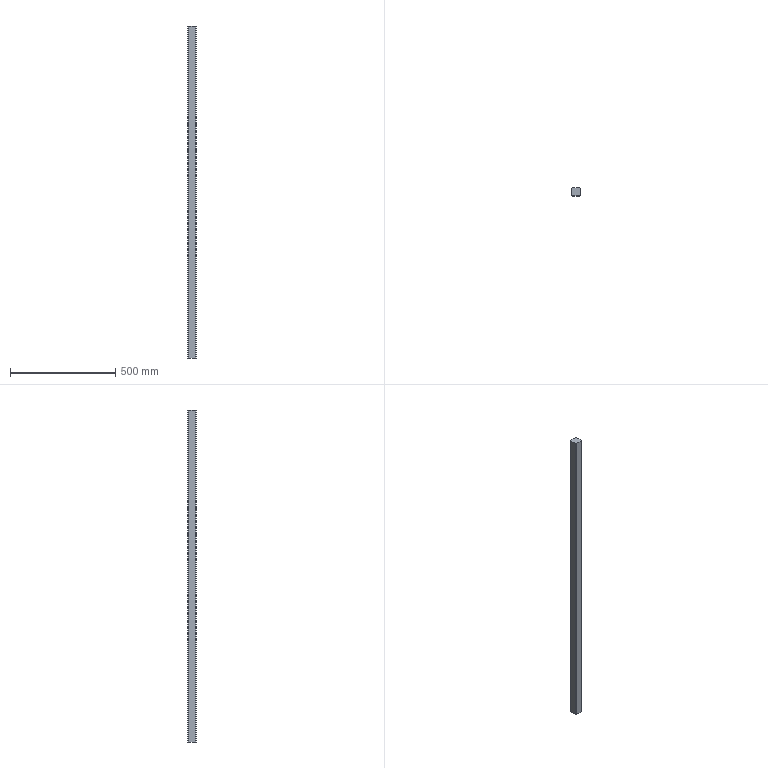Component | SolidWorks | Jig4040-1580-2 | 1 solid | 10 faces | box 40 x 40 x 1580 mm | volume 2494093 mm3 | plane 6 | cylinder 4 | commonest cylinder face diameters 10 x4 | material Copper
build123d program:
from build123d import *

# Parameters (mm, degrees)
SKETCH1_W           = 40
SKETCH1_H           = 40
BOSS_EXTRUDE1_DEPTH = 1580
FILLET1_R           = 5


with BuildPart() as part:
    # Sketch1 → Boss-Extrude1 (new body)
    with BuildSketch(Plane.XY):
        with Locations((20, 20)):
            Rectangle(SKETCH1_W, SKETCH1_H)
    extrude(amount=BOSS_EXTRUDE1_DEPTH)

    # Fillet1
    fillet1_edges = [part.edges().sort_by_distance(p)[0] for p in [
        (0, 40, 790),
        (40, 40, 790),
        (40, 0, 790),
        (0, 0, 790),
    ]]
    fillet(fillet1_edges, radius=FILLET1_R)


solid = part.part

# Placed as in the assembly
solid = solid.moved(Location((711.992, -17.909, 790), (0, 0, 0)))
STEP:
#1=CARTESIAN_POINT('',(28.031,0.6729,31.102));
#2=VERTEX_POINT('',#1);
#3=CARTESIAN_POINT('',(28.031,-0.5082,31.102));
#4=VERTEX_POINT('',#3);
#5=CARTESIAN_POINT('',(28.031,-0.7051,31.102));
#6=DIRECTION('',(0.,-1.,0.));
#7=VECTOR('',#6,39.37);
#8=LINE('',#5,#7);
#9=EDGE_CURVE('',#2,#4,#8,.T.);
#10=ORIENTED_EDGE('',*,*,#9,.T.);
#11=CARTESIAN_POINT('',(28.031,-0.5082,93.307));
#12=VERTEX_POINT('',#11);
#13=CARTESIAN_POINT('',(28.031,-0.5082,93.307));
#14=DIRECTION('',(0.,0.,1.));
#15=VECTOR('',#14,39.37);
#16=LINE('',#13,#15);
#17=EDGE_CURVE('',#4,#12,#16,.T.);
#18=ORIENTED_EDGE('',*,*,#17,.T.);
#19=CARTESIAN_POINT('',(28.031,0.6729,93.307));
#20=VERTEX_POINT('',#19);
#21=CARTESIAN_POINT('',(28.031,-0.7051,93.307));
#22=DIRECTION('',(0.,-1.,0.));
#23=VECTOR('',#22,39.37);
#24=LINE('',#21,#23);
#25=EDGE_CURVE('',#20,#12,#24,.T.);
#26=ORIENTED_EDGE('',*,*,#25,.F.);
#27=CARTESIAN_POINT('',(28.031,0.6729,93.307));
#28=DIRECTION('',(0.,0.,-1.));
#29=VECTOR('',#28,39.37);
#30=LINE('',#27,#29);
#31=EDGE_CURVE('',#20,#2,#30,.T.);
#32=ORIENTED_EDGE('',*,*,#31,.T.);
#33=EDGE_LOOP('',(#10,#18,#26,#32));
#34=FACE_OUTER_BOUND('',#33,.T.);
#35=CARTESIAN_POINT('',(28.031,-0.7051,93.307));
#36=DIRECTION('',(1.,0.,0.));
#37=DIRECTION('',(0.,0.,-1.));
#38=AXIS2_PLACEMENT_3D('',#35,#36,#37);
#39=PLANE('',#38);
#40=ADVANCED_FACE('',(#34),#39,.F.);
#41=CARTESIAN_POINT('',(28.228,-0.7051,93.307));
#42=VERTEX_POINT('',#41);
#43=CARTESIAN_POINT('',(29.409,-0.7051,93.307));
#44=VERTEX_POINT('',#43);
#45=CARTESIAN_POINT('',(28.031,-0.7051,93.307));
#46=DIRECTION('',(1.,0.,0.));
#47=VECTOR('',#46,39.37);
#48=LINE('',#45,#47);
#49=EDGE_CURVE('',#42,#44,#48,.T.);
#50=ORIENTED_EDGE('',*,*,#49,.F.);
#51=CARTESIAN_POINT('',(28.228,-0.7051,31.102));
#52=VERTEX_POINT('',#51);
#53=CARTESIAN_POINT('',(28.228,-0.7051,93.307));
#54=DIRECTION('',(0.,0.,-1.));
#55=VECTOR('',#54,39.37);
#56=LINE('',#53,#55);
#57=EDGE_CURVE('',#42,#52,#56,.T.);
#58=ORIENTED_EDGE('',*,*,#57,.T.);
#59=CARTESIAN_POINT('',(29.409,-0.7051,31.102));
#60=VERTEX_POINT('',#59);
#61=CARTESIAN_POINT('',(28.031,-0.7051,31.102));
#62=DIRECTION('',(1.,0.,0.));
#63=VECTOR('',#62,39.37);
#64=LINE('',#61,#63);
#65=EDGE_CURVE('',#52,#60,#64,.T.);
#66=ORIENTED_EDGE('',*,*,#65,.T.);
#67=CARTESIAN_POINT('',(29.409,-0.7051,93.307));
#68=DIRECTION('',(0.,0.,1.));
#69=VECTOR('',#68,39.37);
#70=LINE('',#67,#69);
#71=EDGE_CURVE('',#60,#44,#70,.T.);
#72=ORIENTED_EDGE('',*,*,#71,.T.);
#73=EDGE_LOOP('',(#50,#58,#66,#72));
#74=FACE_OUTER_BOUND('',#73,.T.);
#75=CARTESIAN_POINT('',(28.031,-0.7051,93.307));
#76=DIRECTION('',(0.,1.,0.));
#77=DIRECTION('',(0.,0.,1.));
#78=AXIS2_PLACEMENT_3D('',#75,#76,#77);
#79=PLANE('',#78);
#80=ADVANCED_FACE('',(#74),#79,.F.);
#81=CARTESIAN_POINT('',(29.606,-0.5082,93.307));
#82=VERTEX_POINT('',#81);
#83=CARTESIAN_POINT('',(29.606,0.6729,93.307));
#84=VERTEX_POINT('',#83);
#85=CARTESIAN_POINT('',(29.606,-0.7051,93.307));
#86=DIRECTION('',(0.,1.,0.));
#87=VECTOR('',#86,39.37);
#88=LINE('',#85,#87);
#89=EDGE_CURVE('',#82,#84,#88,.T.);
#90=ORIENTED_EDGE('',*,*,#89,.F.);
#91=CARTESIAN_POINT('',(29.606,-0.5082,31.102));
#92=VERTEX_POINT('',#91);
#93=CARTESIAN_POINT('',(29.606,-0.5082,93.307));
#94=DIRECTION('',(0.,0.,-1.));
#95=VECTOR('',#94,39.37);
#96=LINE('',#93,#95);
#97=EDGE_CURVE('',#82,#92,#96,.T.);
#98=ORIENTED_EDGE('',*,*,#97,.T.);
#99=CARTESIAN_POINT('',(29.606,0.6729,31.102));
#100=VERTEX_POINT('',#99);
#101=CARTESIAN_POINT('',(29.606,-0.7051,31.102));
#102=DIRECTION('',(0.,1.,0.));
#103=VECTOR('',#102,39.37);
#104=LINE('',#101,#103);
#105=EDGE_CURVE('',#92,#100,#104,.T.);
#106=ORIENTED_EDGE('',*,*,#105,.T.);
#107=CARTESIAN_POINT('',(29.606,0.6729,93.307));
#108=DIRECTION('',(0.,0.,1.));
#109=VECTOR('',#108,39.37);
#110=LINE('',#107,#109);
#111=EDGE_CURVE('',#100,#84,#110,.T.);
#112=ORIENTED_EDGE('',*,*,#111,.T.);
#113=EDGE_LOOP('',(#90,#98,#106,#112));
#114=FACE_OUTER_BOUND('',#113,.T.);
#115=CARTESIAN_POINT('',(29.606,-0.7051,93.307));
#116=DIRECTION('',(-1.,0.,0.));
#117=DIRECTION('',(0.,0.,1.));
#118=AXIS2_PLACEMENT_3D('',#115,#116,#117);
#119=PLANE('',#118);
#120=ADVANCED_FACE('',(#114),#119,.F.);
#121=CARTESIAN_POINT('',(29.409,0.8697,31.102));
#122=VERTEX_POINT('',#121);
#123=CARTESIAN_POINT('',(28.228,0.8697,31.102));
#124=VERTEX_POINT('',#123);
#125=CARTESIAN_POINT('',(28.031,0.8697,31.102));
#126=DIRECTION('',(-1.,0.,0.));
#127=VECTOR('',#126,39.37);
#128=LINE('',#125,#127);
#129=EDGE_CURVE('',#122,#124,#128,.T.);
#130=ORIENTED_EDGE('',*,*,#129,.T.);
#131=CARTESIAN_POINT('',(28.228,0.8697,93.307));
#132=VERTEX_POINT('',#131);
#133=CARTESIAN_POINT('',(28.228,0.8697,93.307));
#134=DIRECTION('',(0.,0.,1.));
#135=VECTOR('',#134,39.37);
#136=LINE('',#133,#135);
#137=EDGE_CURVE('',#124,#132,#136,.T.);
#138=ORIENTED_EDGE('',*,*,#137,.T.);
#139=CARTESIAN_POINT('',(29.409,0.8697,93.307));
#140=VERTEX_POINT('',#139);
#141=CARTESIAN_POINT('',(28.031,0.8697,93.307));
#142=DIRECTION('',(-1.,0.,0.));
#143=VECTOR('',#142,39.37);
#144=LINE('',#141,#143);
#145=EDGE_CURVE('',#140,#132,#144,.T.);
#146=ORIENTED_EDGE('',*,*,#145,.F.);
#147=CARTESIAN_POINT('',(29.409,0.8697,93.307));
#148=DIRECTION('',(0.,0.,-1.));
#149=VECTOR('',#148,39.37);
#150=LINE('',#147,#149);
#151=EDGE_CURVE('',#140,#122,#150,.T.);
#152=ORIENTED_EDGE('',*,*,#151,.T.);
#153=EDGE_LOOP('',(#130,#138,#146,#152));
#154=FACE_OUTER_BOUND('',#153,.T.);
#155=CARTESIAN_POINT('',(28.031,0.8697,93.307));
#156=DIRECTION('',(0.,-1.,0.));
#157=DIRECTION('',(0.,0.,-1.));
#158=AXIS2_PLACEMENT_3D('',#155,#156,#157);
#159=PLANE('',#158);
#160=ADVANCED_FACE('',(#154),#159,.F.);
#161=ORIENTED_EDGE('',*,*,#25,.T.);
#162=CARTESIAN_POINT('',(28.228,-0.5082,93.307));
#163=DIRECTION('',(0.,0.,1.));
#164=DIRECTION('',(-1.,0.,0.));
#165=AXIS2_PLACEMENT_3D('',#162,#163,#164);
#166=CIRCLE('',#165,0.1969);
#167=EDGE_CURVE('',#12,#42,#166,.T.);
#168=ORIENTED_EDGE('',*,*,#167,.T.);
#169=ORIENTED_EDGE('',*,*,#49,.T.);
#170=CARTESIAN_POINT('',(29.409,-0.5082,93.307));
#171=DIRECTION('',(0.,0.,1.));
#172=DIRECTION('',(-1.,0.,0.));
#173=AXIS2_PLACEMENT_3D('',#170,#171,#172);
#174=CIRCLE('',#173,0.1969);
#175=EDGE_CURVE('',#44,#82,#174,.T.);
#176=ORIENTED_EDGE('',*,*,#175,.T.);
#177=ORIENTED_EDGE('',*,*,#89,.T.);
#178=CARTESIAN_POINT('',(29.409,0.6729,93.307));
#179=DIRECTION('',(0.,0.,1.));
#180=DIRECTION('',(-1.,0.,0.));
#181=AXIS2_PLACEMENT_3D('',#178,#179,#180);
#182=CIRCLE('',#181,0.1969);
#183=EDGE_CURVE('',#84,#140,#182,.T.);
#184=ORIENTED_EDGE('',*,*,#183,.T.);
#185=ORIENTED_EDGE('',*,*,#145,.T.);
#186=CARTESIAN_POINT('',(28.228,0.6729,93.307));
#187=DIRECTION('',(0.,0.,1.));
#188=DIRECTION('',(-1.,0.,0.));
#189=AXIS2_PLACEMENT_3D('',#186,#187,#188);
#190=CIRCLE('',#189,0.1969);
#191=EDGE_CURVE('',#132,#20,#190,.T.);
#192=ORIENTED_EDGE('',*,*,#191,.T.);
#193=EDGE_LOOP('',(#161,#168,#169,#176,#177,#184,#185,#192));
#194=FACE_OUTER_BOUND('',#193,.T.);
#195=CARTESIAN_POINT('',(28.031,-0.7051,93.307));
#196=DIRECTION('',(0.,0.,-1.));
#197=DIRECTION('',(-1.,0.,0.));
#198=AXIS2_PLACEMENT_3D('',#195,#196,#197);
#199=PLANE('',#198);
#200=ADVANCED_FACE('',(#194),#199,.F.);
#201=ORIENTED_EDGE('',*,*,#65,.F.);
#202=CARTESIAN_POINT('',(28.228,-0.5082,31.102));
#203=DIRECTION('',(0.,0.,-1.));
#204=DIRECTION('',(-1.,0.,0.));
#205=AXIS2_PLACEMENT_3D('',#202,#203,#204);
#206=CIRCLE('',#205,0.1969);
#207=EDGE_CURVE('',#52,#4,#206,.T.);
#208=ORIENTED_EDGE('',*,*,#207,.T.);
#209=ORIENTED_EDGE('',*,*,#9,.F.);
#210=CARTESIAN_POINT('',(28.228,0.6729,31.102));
#211=DIRECTION('',(0.,0.,-1.));
#212=DIRECTION('',(-1.,0.,0.));
#213=AXIS2_PLACEMENT_3D('',#210,#211,#212);
#214=CIRCLE('',#213,0.1969);
#215=EDGE_CURVE('',#2,#124,#214,.T.);
#216=ORIENTED_EDGE('',*,*,#215,.T.);
#217=ORIENTED_EDGE('',*,*,#129,.F.);
#218=CARTESIAN_POINT('',(29.409,0.6729,31.102));
#219=DIRECTION('',(0.,0.,-1.));
#220=DIRECTION('',(-1.,0.,0.));
#221=AXIS2_PLACEMENT_3D('',#218,#219,#220);
#222=CIRCLE('',#221,0.1969);
#223=EDGE_CURVE('',#122,#100,#222,.T.);
#224=ORIENTED_EDGE('',*,*,#223,.T.);
#225=ORIENTED_EDGE('',*,*,#105,.F.);
#226=CARTESIAN_POINT('',(29.409,-0.5082,31.102));
#227=DIRECTION('',(0.,0.,-1.));
#228=DIRECTION('',(-1.,0.,0.));
#229=AXIS2_PLACEMENT_3D('',#226,#227,#228);
#230=CIRCLE('',#229,0.1969);
#231=EDGE_CURVE('',#92,#60,#230,.T.);
#232=ORIENTED_EDGE('',*,*,#231,.T.);
#233=EDGE_LOOP('',(#201,#208,#209,#216,#217,#224,#225,#232));
#234=FACE_OUTER_BOUND('',#233,.T.);
#235=CARTESIAN_POINT('',(28.031,-0.7051,31.102));
#236=DIRECTION('',(0.,0.,-1.));
#237=DIRECTION('',(-1.,0.,0.));
#238=AXIS2_PLACEMENT_3D('',#235,#236,#237);
#239=PLANE('',#238);
#240=ADVANCED_FACE('',(#234),#239,.T.);
#241=ORIENTED_EDGE('',*,*,#167,.F.);
#242=ORIENTED_EDGE('',*,*,#17,.F.);
#243=ORIENTED_EDGE('',*,*,#207,.F.);
#244=ORIENTED_EDGE('',*,*,#57,.F.);
#245=EDGE_LOOP('',(#241,#242,#243,#244));
#246=FACE_OUTER_BOUND('',#245,.T.);
#247=CARTESIAN_POINT('',(28.228,-0.5082,93.307));
#248=DIRECTION('',(0.,0.,-1.));
#249=DIRECTION('',(-1.,0.,0.));
#250=AXIS2_PLACEMENT_3D('',#247,#248,#249);
#251=CYLINDRICAL_SURFACE('',#250,0.1969);
#252=ADVANCED_FACE('',(#246),#251,.T.);
#253=ORIENTED_EDGE('',*,*,#191,.F.);
#254=ORIENTED_EDGE('',*,*,#137,.F.);
#255=ORIENTED_EDGE('',*,*,#215,.F.);
#256=ORIENTED_EDGE('',*,*,#31,.F.);
#257=EDGE_LOOP('',(#253,#254,#255,#256));
#258=FACE_OUTER_BOUND('',#257,.T.);
#259=CARTESIAN_POINT('',(28.228,0.6729,93.307));
#260=DIRECTION('',(0.,0.,-1.));
#261=DIRECTION('',(-1.,0.,0.));
#262=AXIS2_PLACEMENT_3D('',#259,#260,#261);
#263=CYLINDRICAL_SURFACE('',#262,0.1969);
#264=ADVANCED_FACE('',(#258),#263,.T.);
#265=ORIENTED_EDGE('',*,*,#175,.F.);
#266=ORIENTED_EDGE('',*,*,#71,.F.);
#267=ORIENTED_EDGE('',*,*,#231,.F.);
#268=ORIENTED_EDGE('',*,*,#97,.F.);
#269=EDGE_LOOP('',(#265,#266,#267,#268));
#270=FACE_OUTER_BOUND('',#269,.T.);
#271=CARTESIAN_POINT('',(29.409,-0.5082,93.307));
#272=DIRECTION('',(0.,0.,-1.));
#273=DIRECTION('',(-1.,0.,0.));
#274=AXIS2_PLACEMENT_3D('',#271,#272,#273);
#275=CYLINDRICAL_SURFACE('',#274,0.1969);
#276=ADVANCED_FACE('',(#270),#275,.T.);
#277=ORIENTED_EDGE('',*,*,#183,.F.);
#278=ORIENTED_EDGE('',*,*,#111,.F.);
#279=ORIENTED_EDGE('',*,*,#223,.F.);
#280=ORIENTED_EDGE('',*,*,#151,.F.);
#281=EDGE_LOOP('',(#277,#278,#279,#280));
#282=FACE_OUTER_BOUND('',#281,.T.);
#283=CARTESIAN_POINT('',(29.409,0.6729,93.307));
#284=DIRECTION('',(0.,0.,-1.));
#285=DIRECTION('',(-1.,0.,0.));
#286=AXIS2_PLACEMENT_3D('',#283,#284,#285);
#287=CYLINDRICAL_SURFACE('',#286,0.1969);
#288=ADVANCED_FACE('',(#282),#287,.T.);
#289=CLOSED_SHELL('',(#40,#80,#120,#160,#200,#240,#252,#264,#276,#288));
#290=MANIFOLD_SOLID_BREP('',#289);
#291=CARTESIAN_POINT('',(0.,0.,0.));
#292=DIRECTION('',(0.,0.,1.));
#293=DIRECTION('',(1.,0.,0.));
#294=AXIS2_PLACEMENT_3D('',#291,#292,#293);
#295=(LENGTH_UNIT()NAMED_UNIT(*)SI_UNIT($,.METRE.));
#296=LENGTH_MEASURE_WITH_UNIT(LENGTH_MEASURE(0.0254),#295);
#297=DIMENSIONAL_EXPONENTS(1.,0.,0.,0.,0.,0.,0.);
#298=(CONVERSION_BASED_UNIT('',#296)LENGTH_UNIT()NAMED_UNIT(#297));
#299=UNCERTAINTY_MEASURE_WITH_UNIT(LENGTH_MEASURE(0.00001),#298,'','');
#300=(NAMED_UNIT(*)PLANE_ANGLE_UNIT()SI_UNIT($,.RADIAN.));
#301=(NAMED_UNIT(*)SI_UNIT($,.STERADIAN.)SOLID_ANGLE_UNIT());
#302=(GEOMETRIC_REPRESENTATION_CONTEXT(3)GLOBAL_UNCERTAINTY_ASSIGNED_CONTEXT((#299))GLOBAL_UNIT_ASSIGNED_CONTEXT((#298,#300,#301))REPRESENTATION_CONTEXT('',''));
#303=ADVANCED_BREP_SHAPE_REPRESENTATION('',(#290,#294),#302);
#304=COLOUR_RGB('',0.7922,0.8196,0.9333);
#305=FILL_AREA_STYLE_COLOUR('',#304);
#306=FILL_AREA_STYLE('',(#305));
#307=SURFACE_STYLE_FILL_AREA(#306);
#308=SURFACE_SIDE_STYLE('',(#307));
#309=SURFACE_STYLE_USAGE(.BOTH.,#308);
#310=PRESENTATION_STYLE_ASSIGNMENT((#309));
#311=STYLED_ITEM('',(#310),#290);
#312=PRESENTATION_LAYER_ASSIGNMENT('','',(#311));
#313=(LENGTH_UNIT()NAMED_UNIT(*)SI_UNIT($,.METRE.));
#314=LENGTH_MEASURE_WITH_UNIT(LENGTH_MEASURE(0.0254),#313);
#315=DIMENSIONAL_EXPONENTS(1.,0.,0.,0.,0.,0.,0.);
#316=(CONVERSION_BASED_UNIT('',#314)LENGTH_UNIT()NAMED_UNIT(#315));
#317=UNCERTAINTY_MEASURE_WITH_UNIT(LENGTH_MEASURE(0.00001),#316,'','');
#318=(NAMED_UNIT(*)PLANE_ANGLE_UNIT()SI_UNIT($,.RADIAN.));
#319=(NAMED_UNIT(*)SI_UNIT($,.STERADIAN.)SOLID_ANGLE_UNIT());
#320=(GEOMETRIC_REPRESENTATION_CONTEXT(3)GLOBAL_UNCERTAINTY_ASSIGNED_CONTEXT((#317))GLOBAL_UNIT_ASSIGNED_CONTEXT((#316,#318,#319))REPRESENTATION_CONTEXT('',''));
#321=MECHANICAL_DESIGN_GEOMETRIC_PRESENTATION_REPRESENTATION('',(#311),#320);